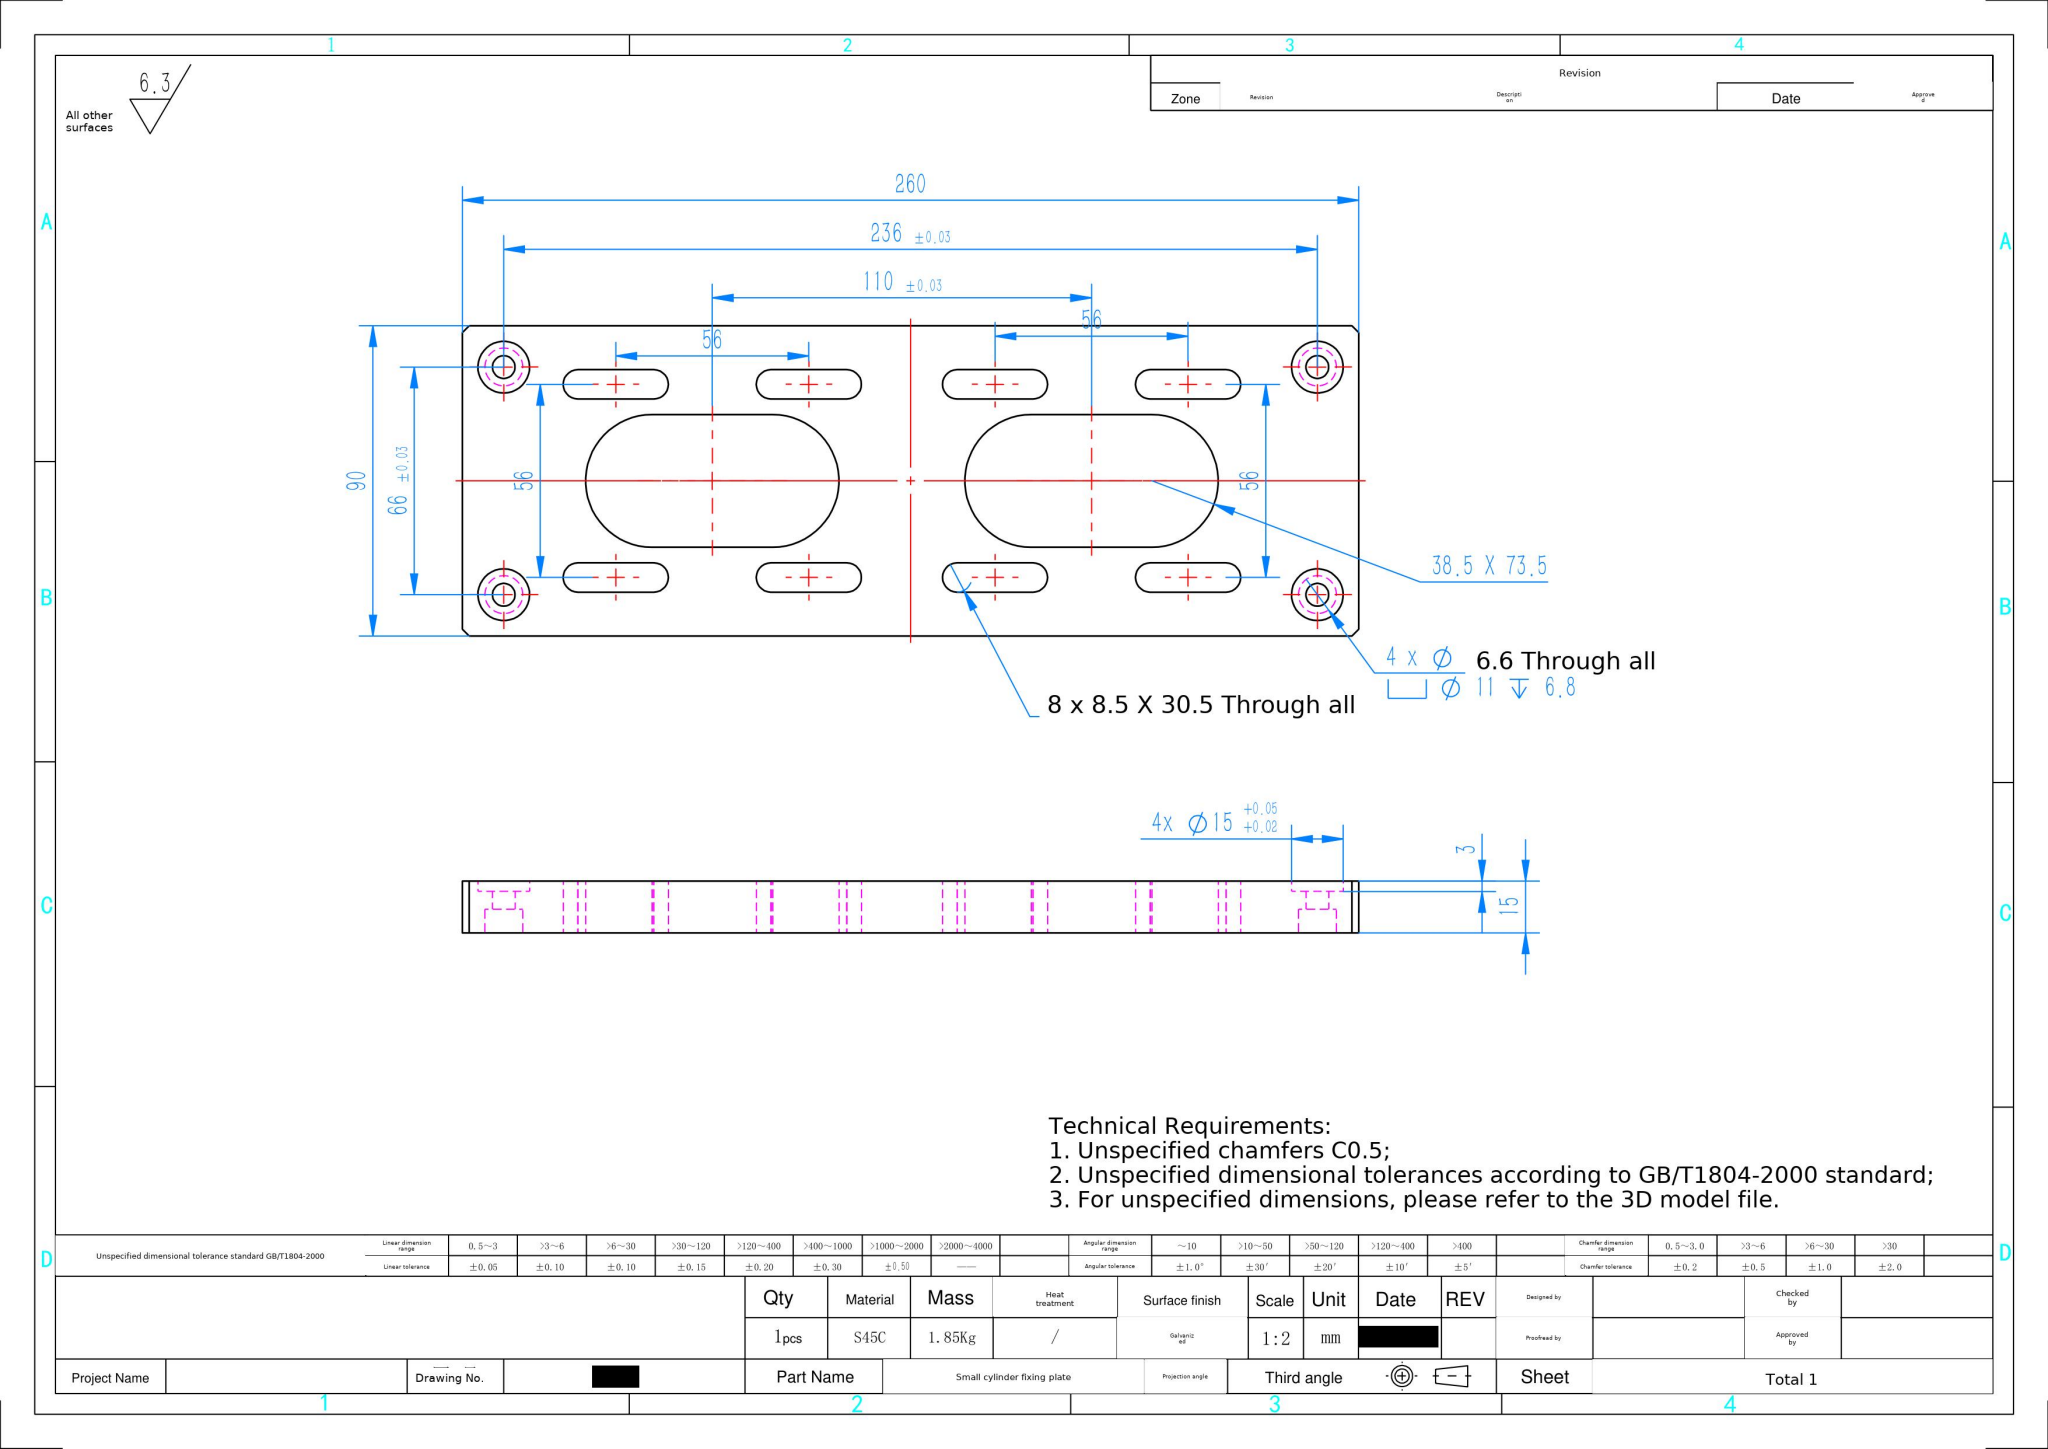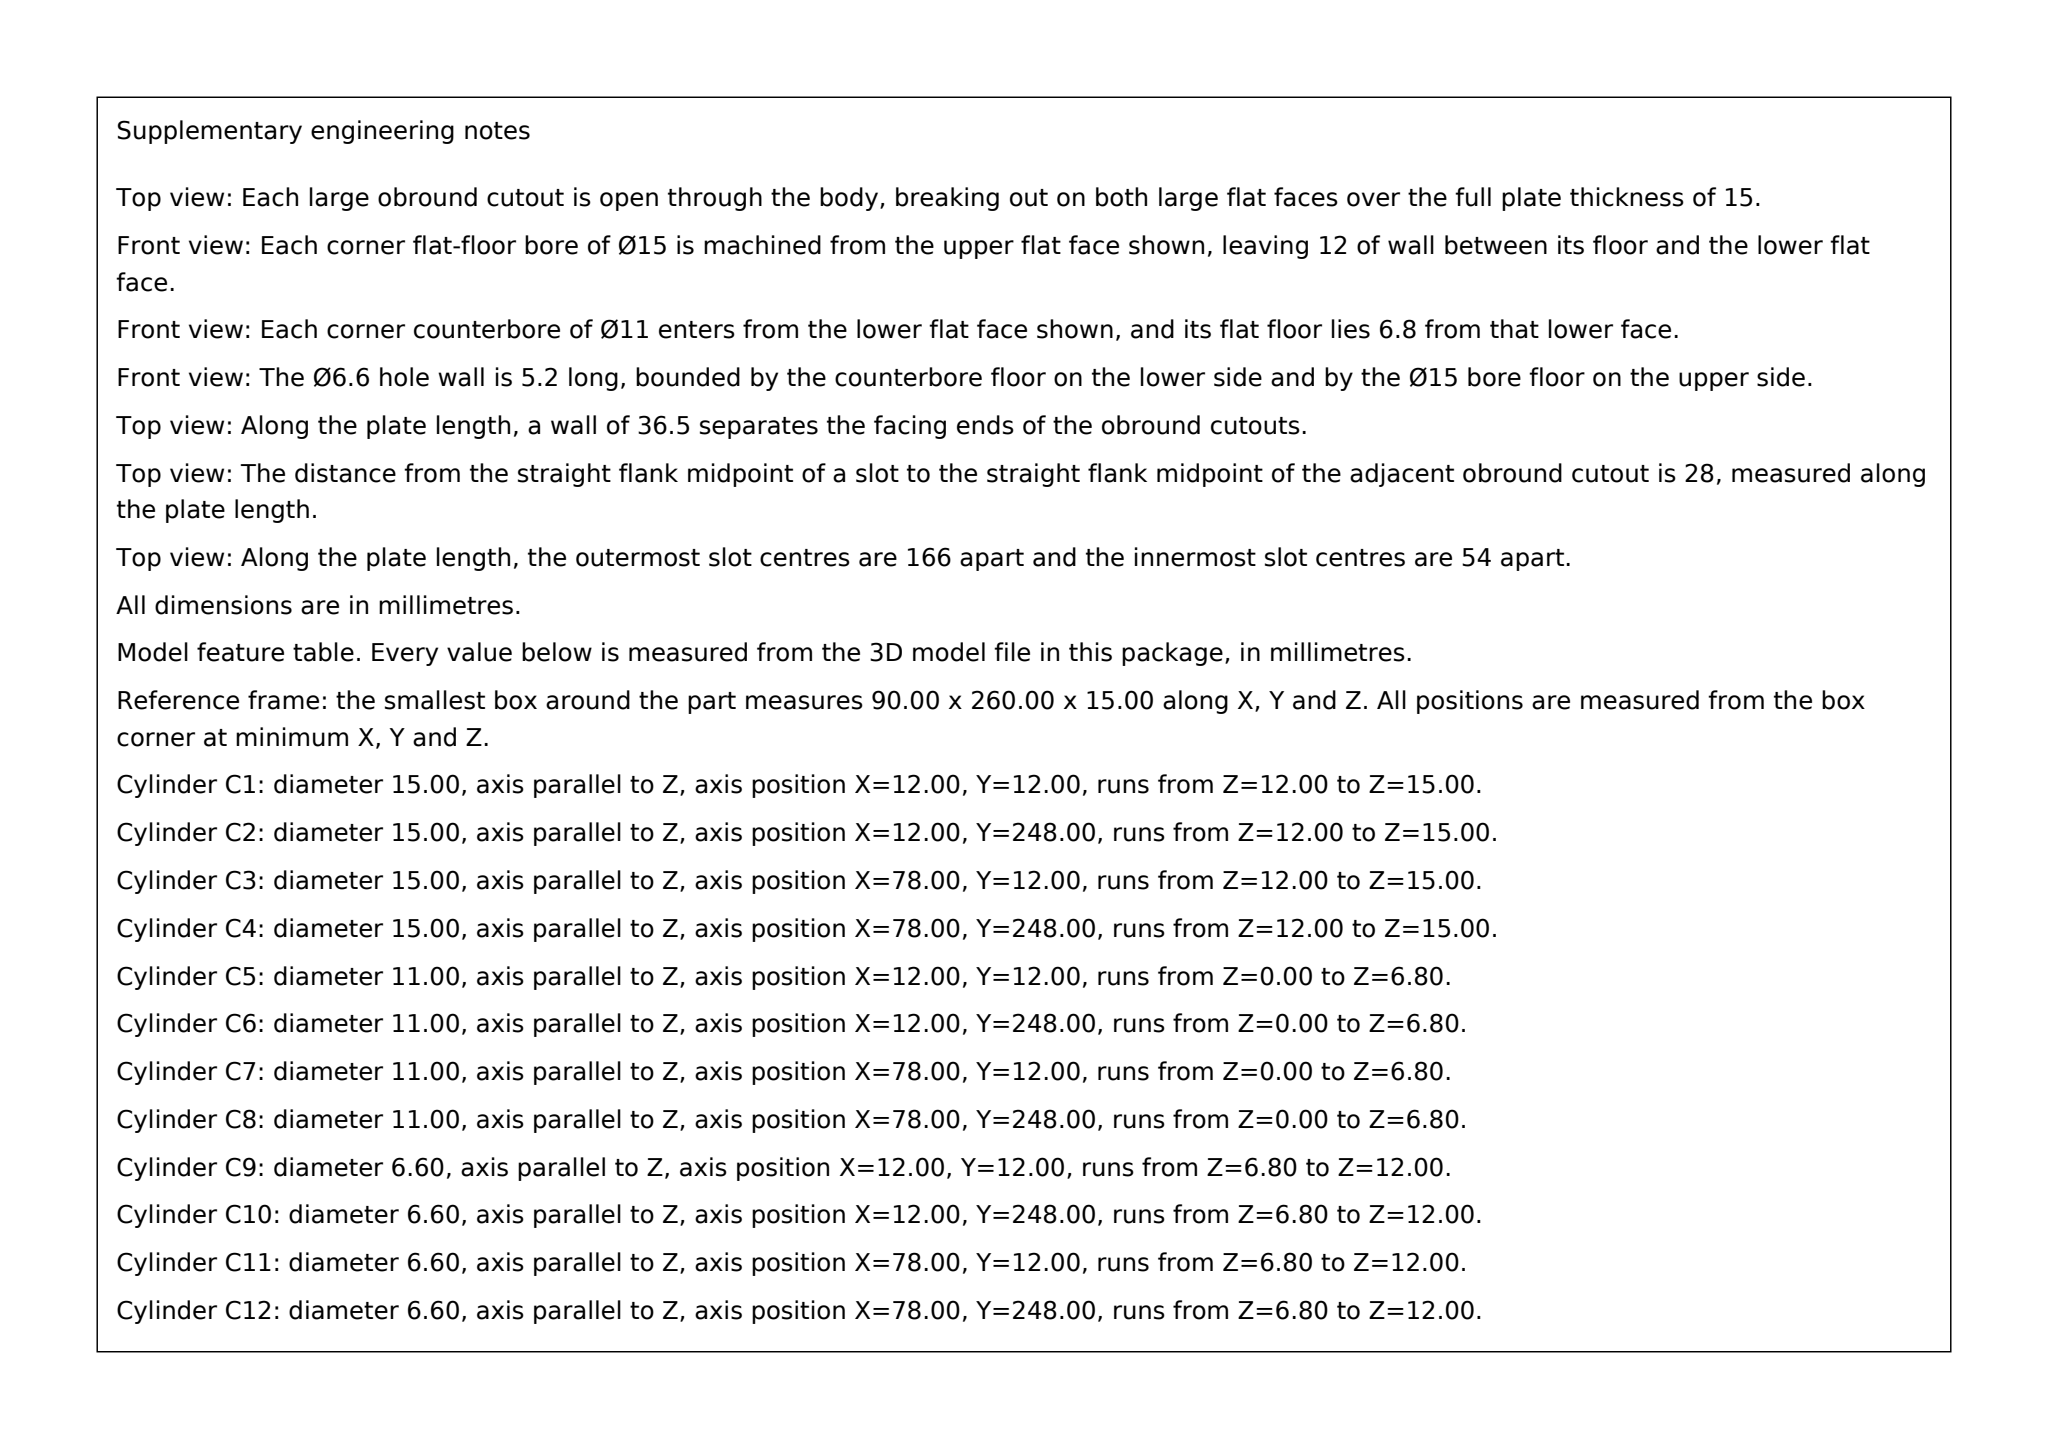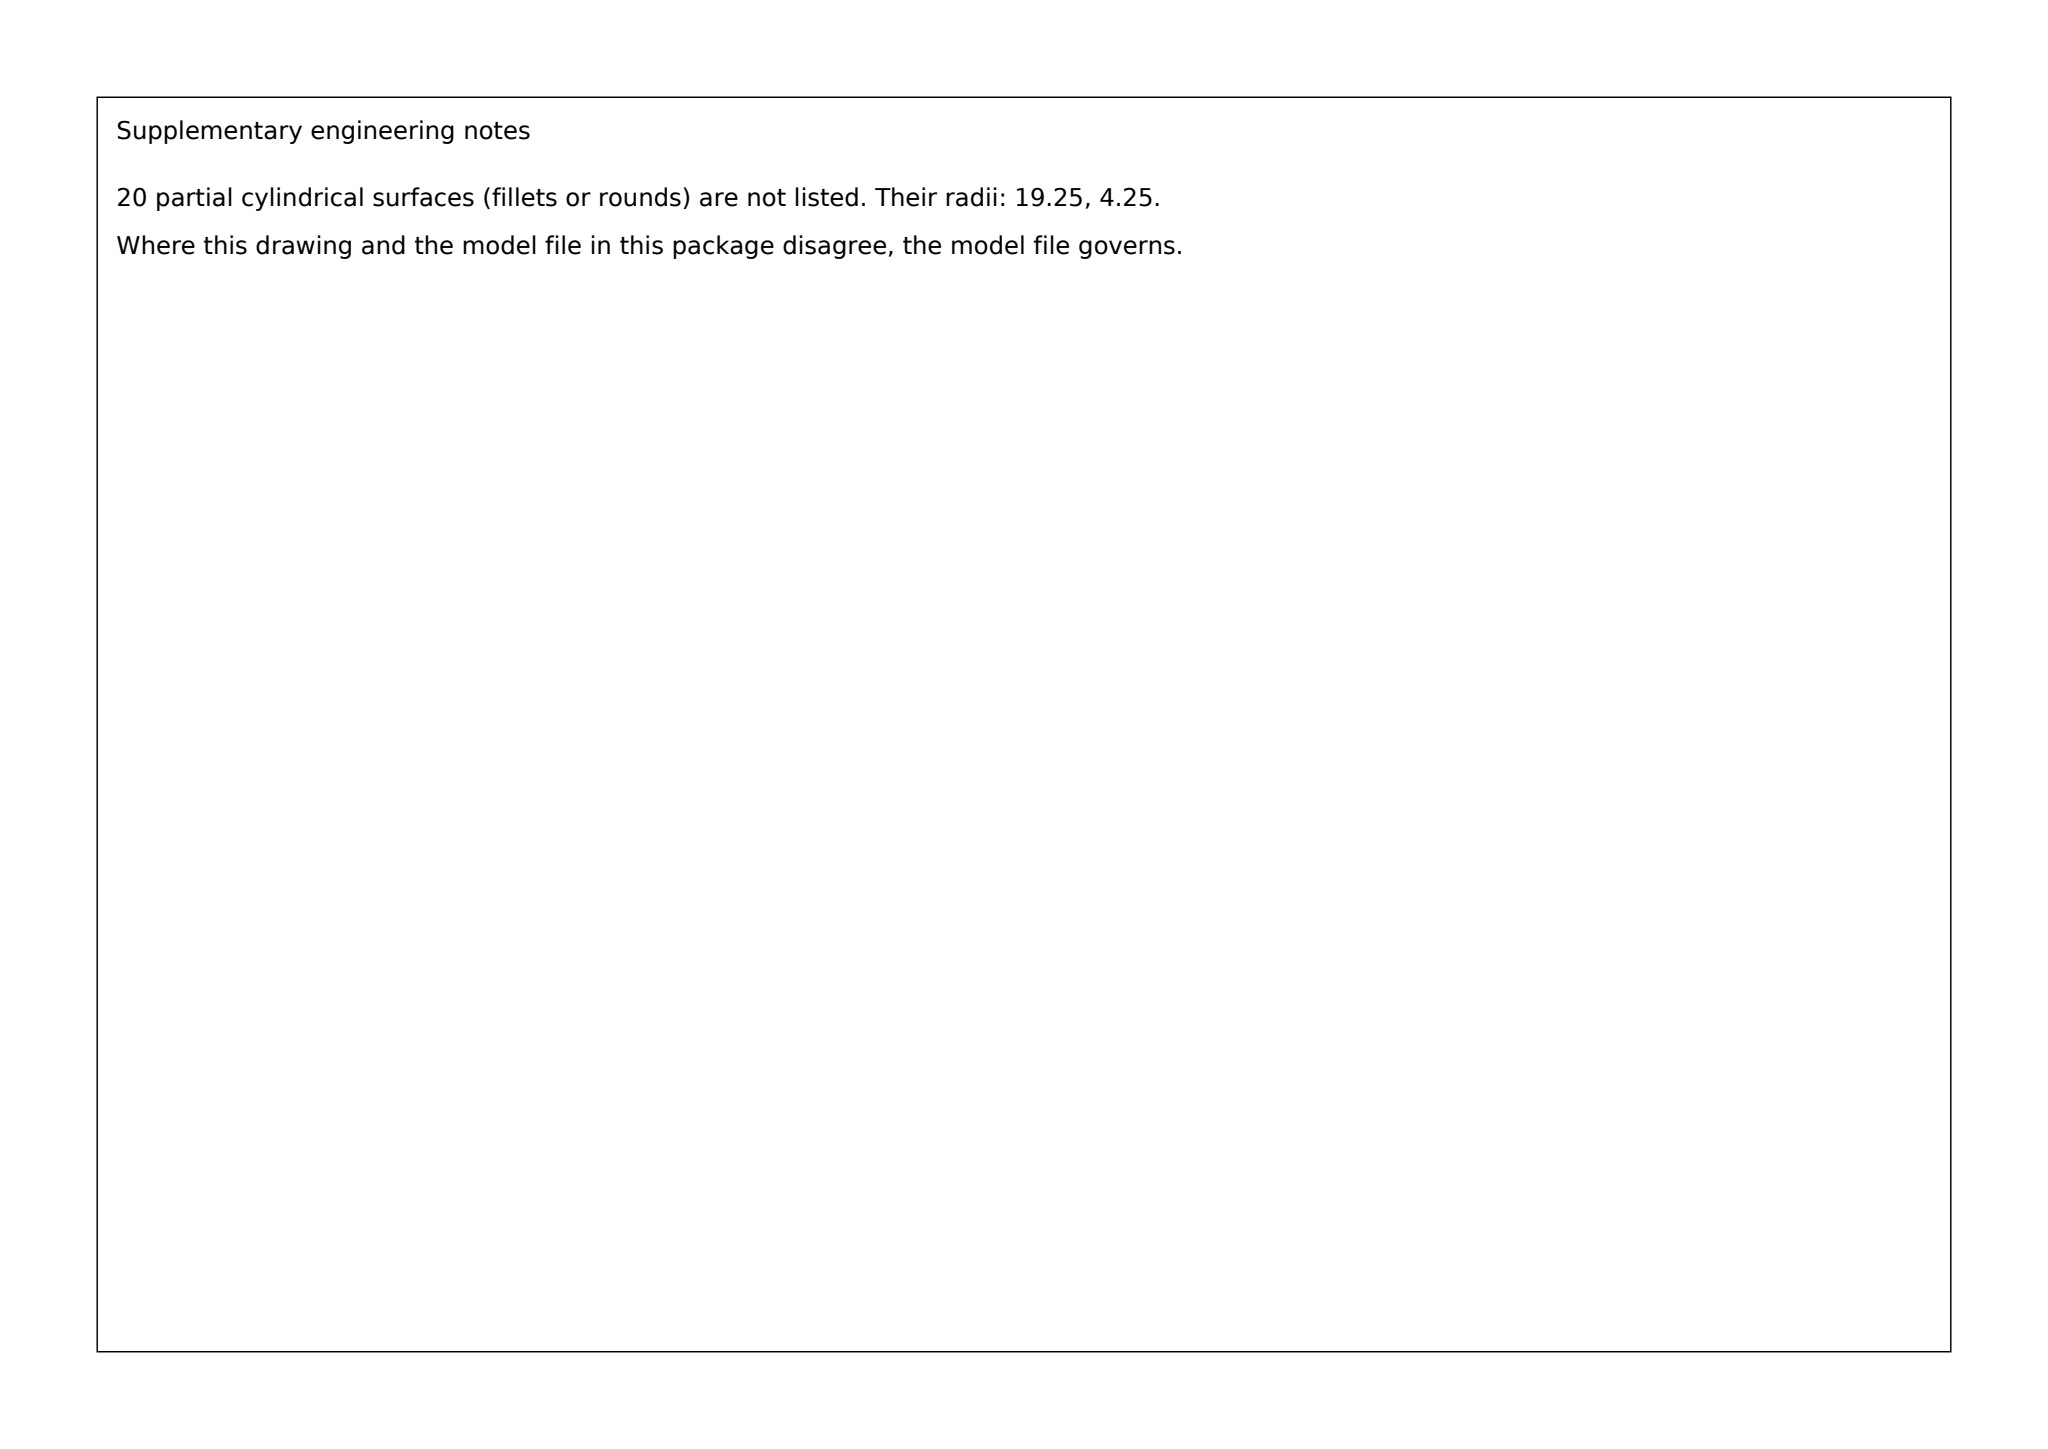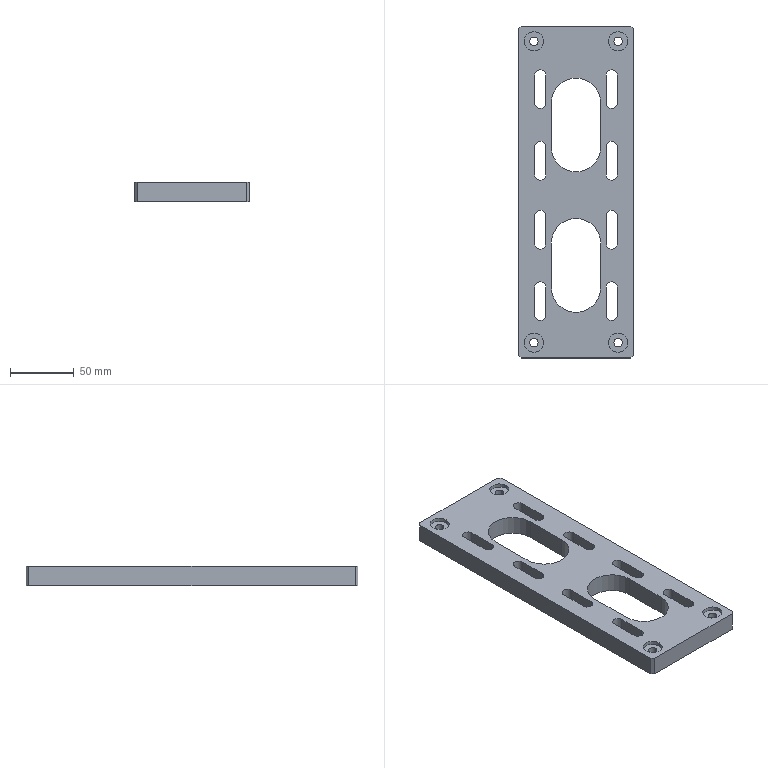Part | SolidWorks | mm | 1 solid | 82 faces | box 90 x 260 x 15 mm | volume 240864 mm3 | cylinder 44 | plane 38 | commonest cylinder face diameters 8.5 x16 11 x8 6.6 x8 15 x8 38.5 x4